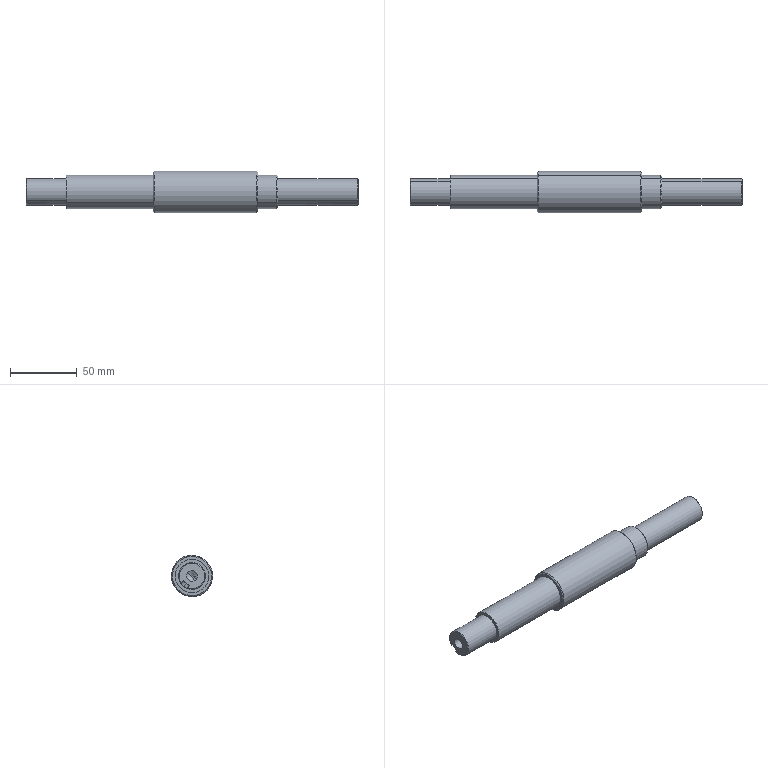Component | SolidWorks | InputAxis-1 | 1 solid | 46 faces | volume 121928 mm3 | cylinder 18 | cone 16 | plane 12 | commonest cylinder face diameters 20 x4 25 x4 6 x4 8 x2 10 x2 31 x2